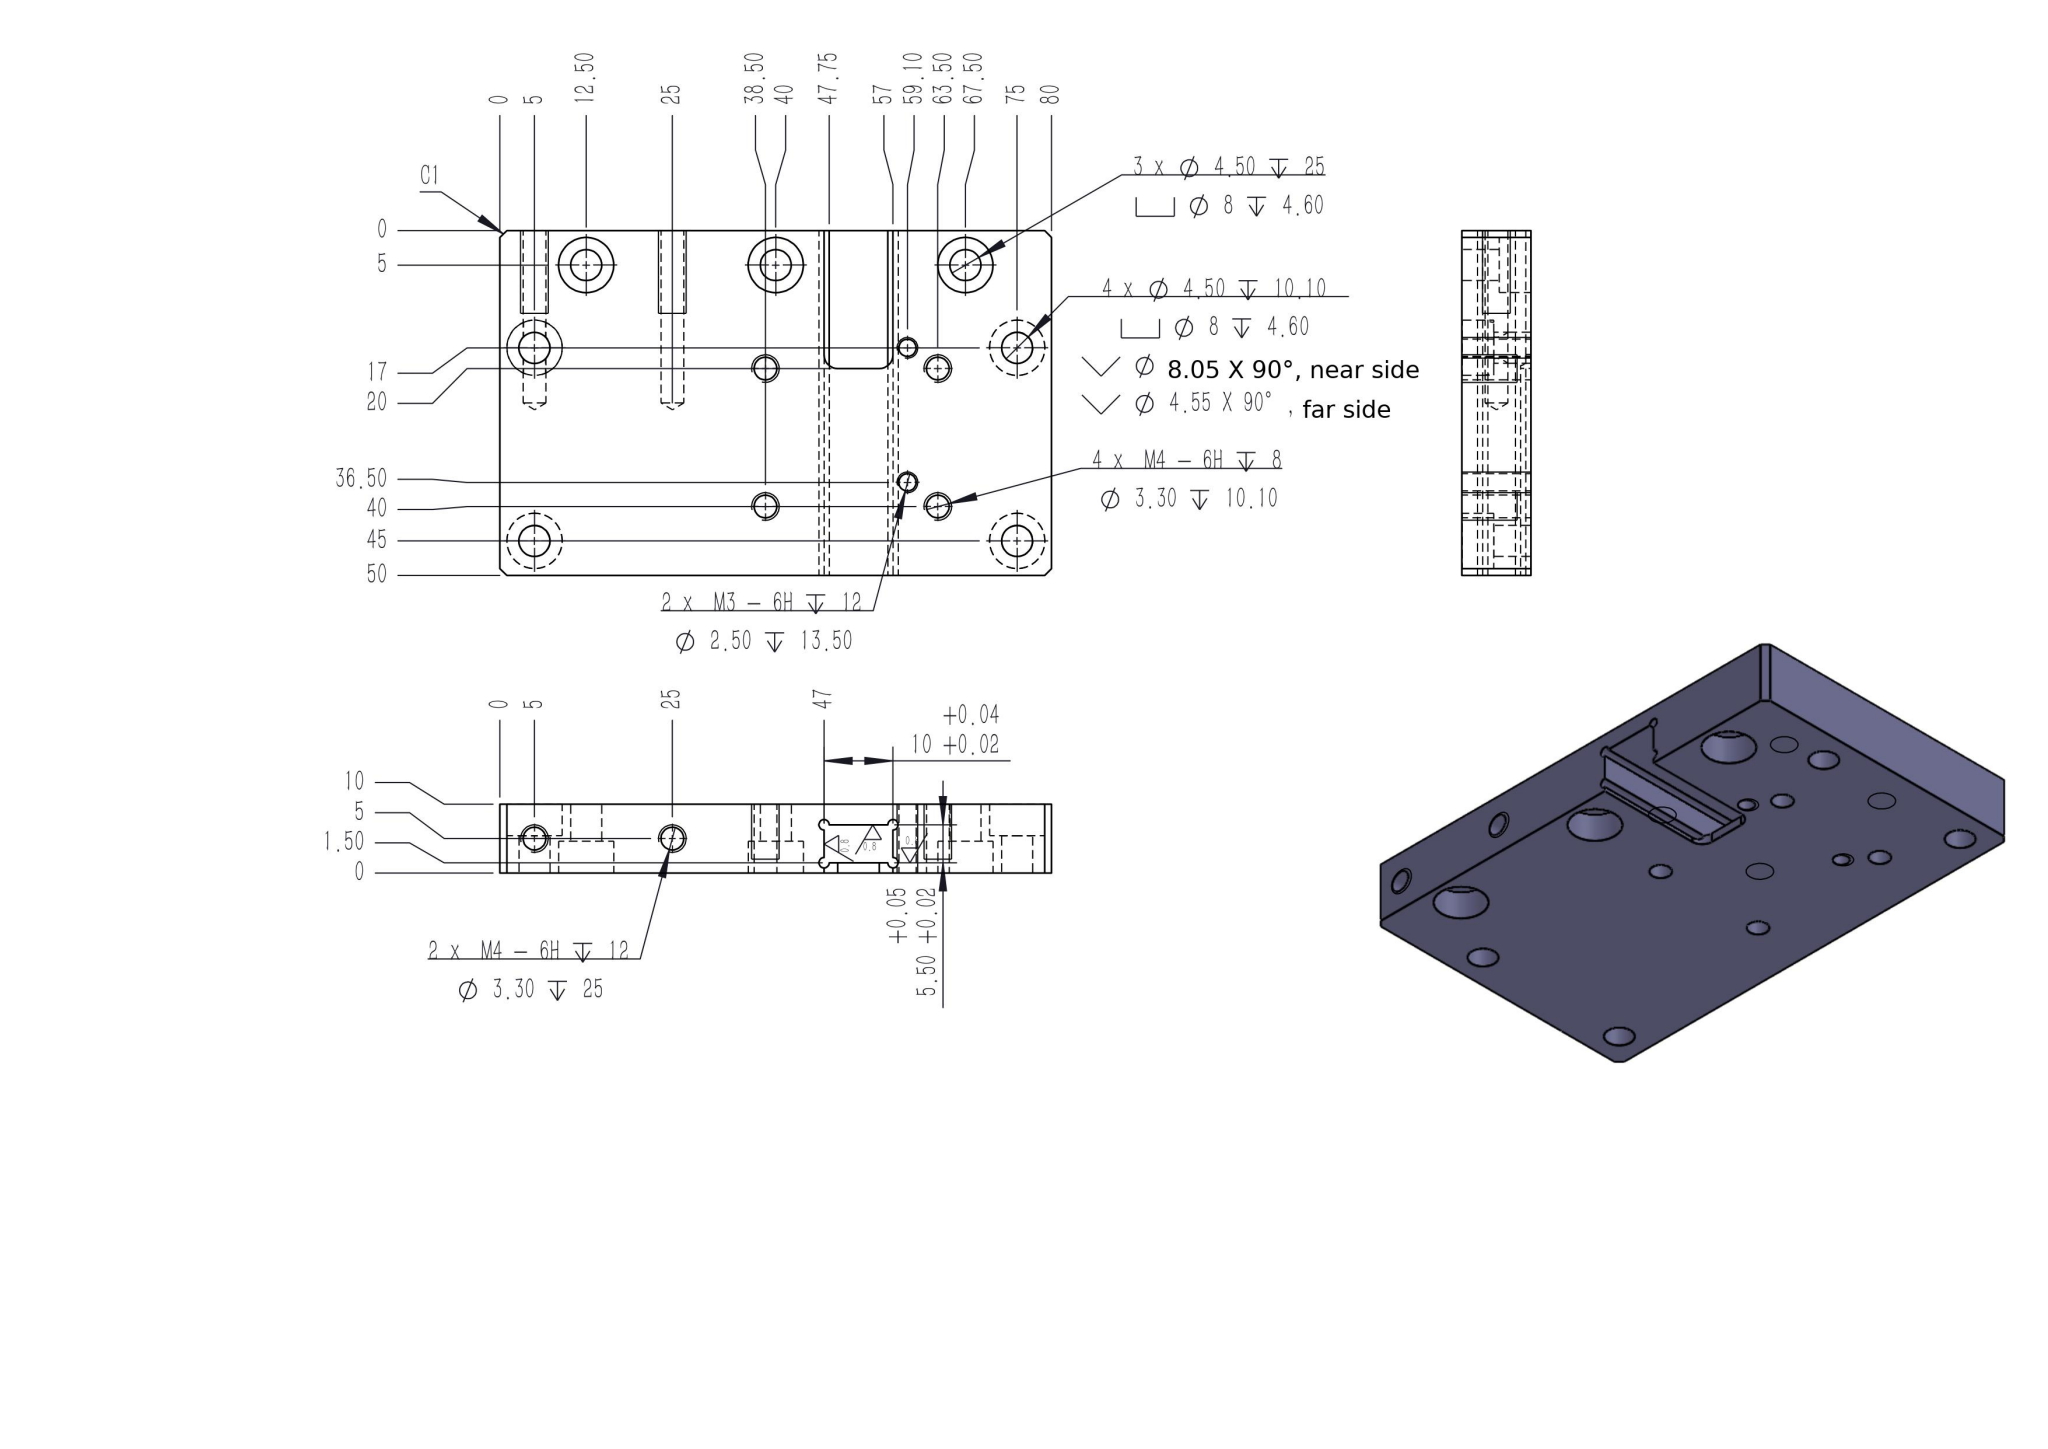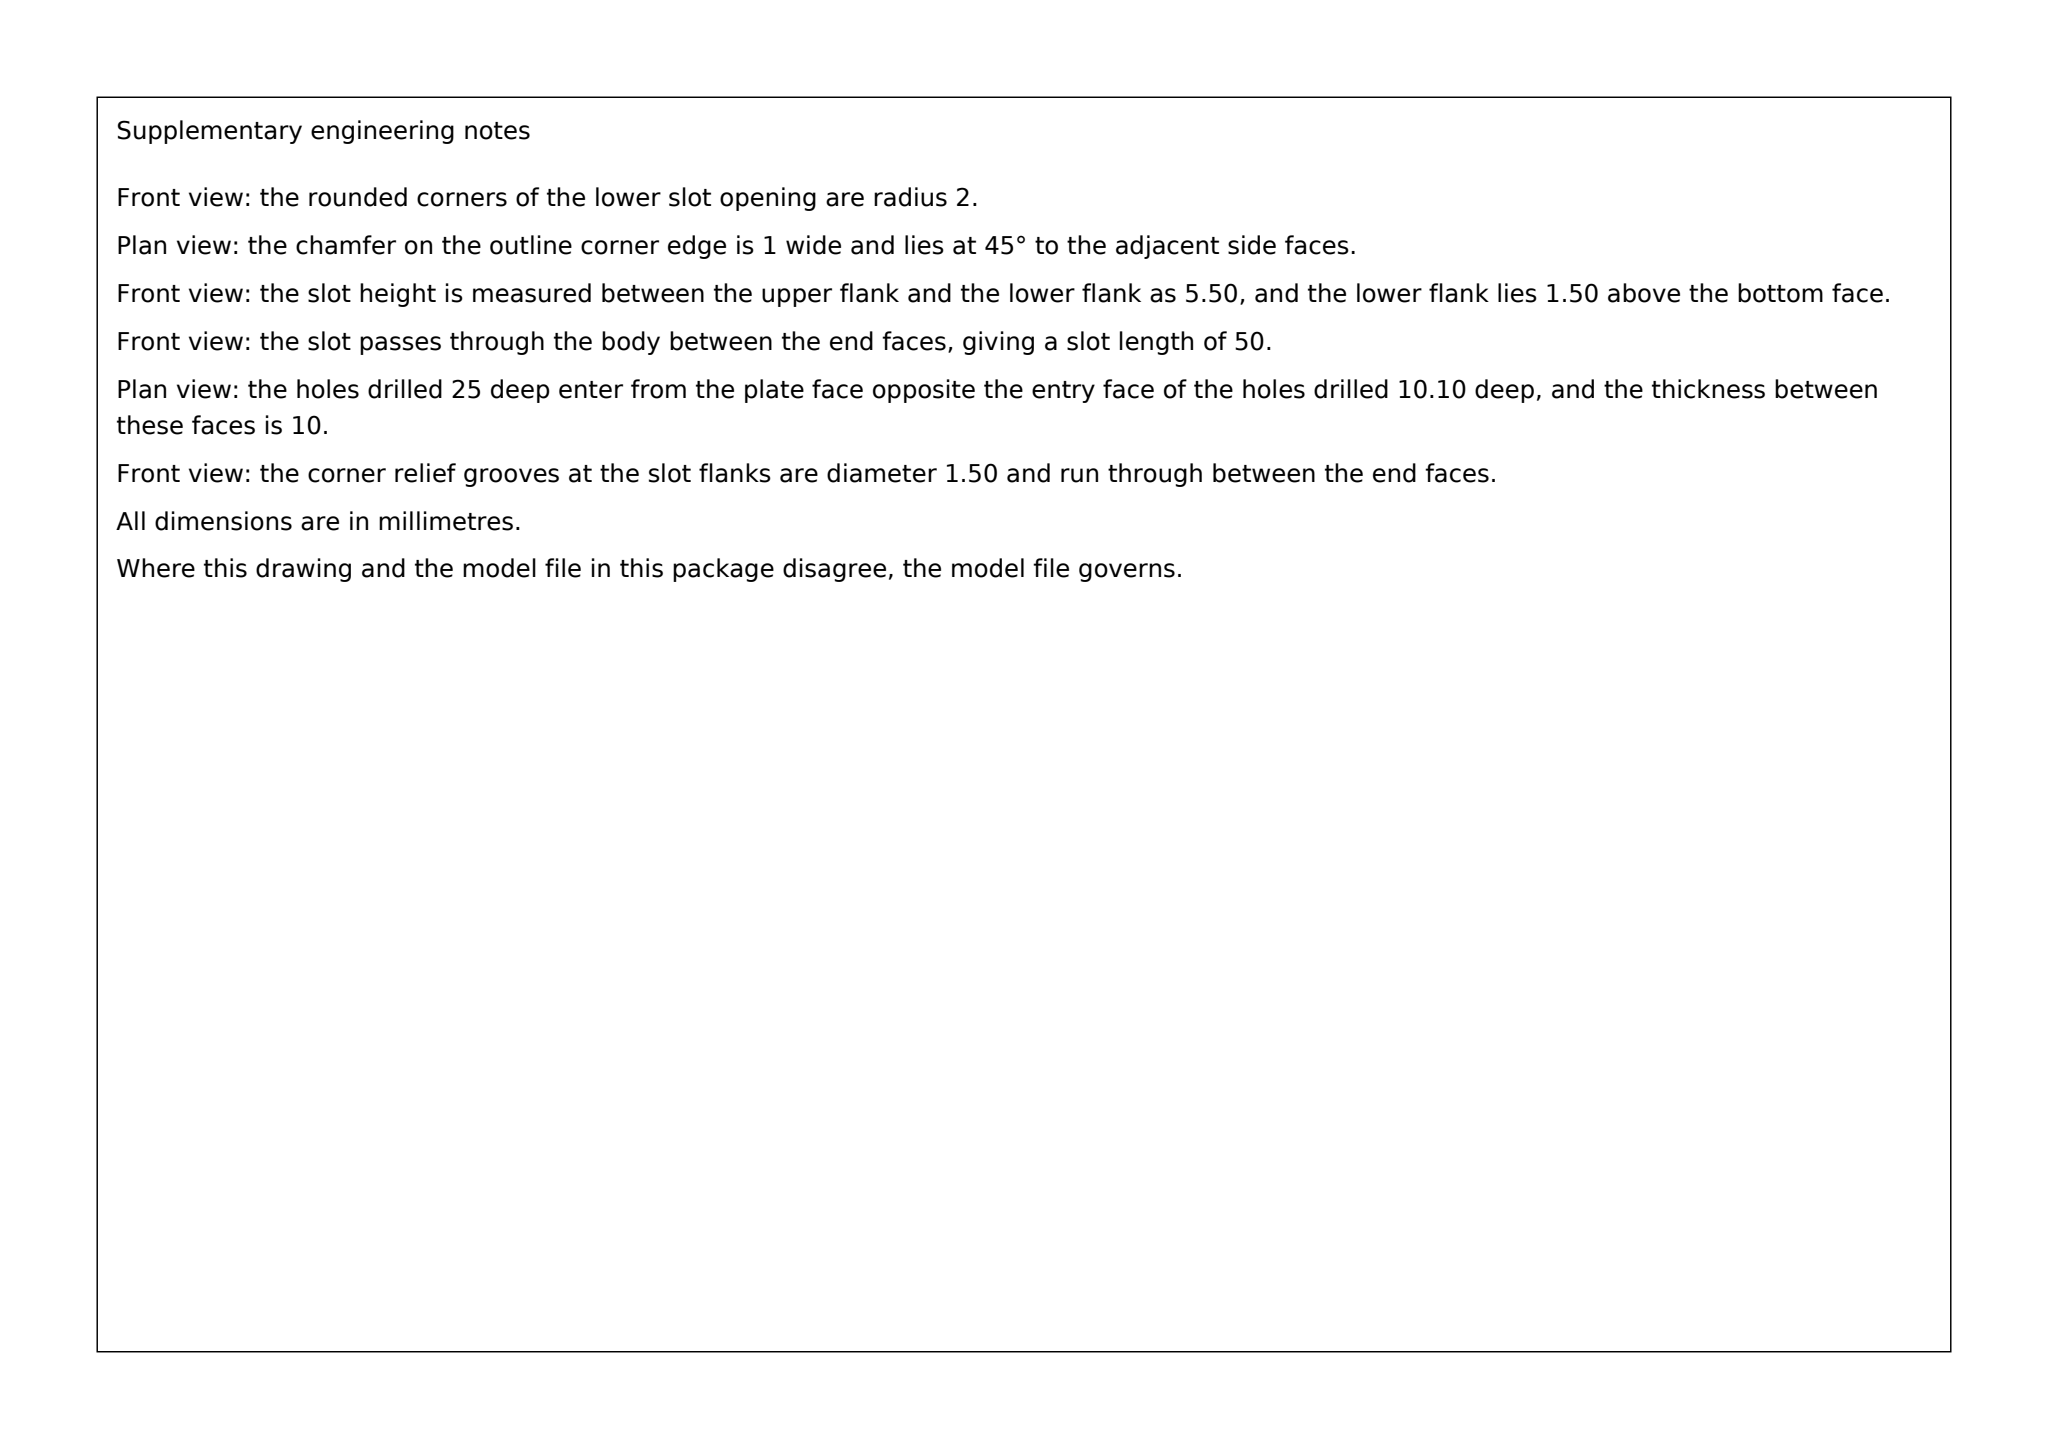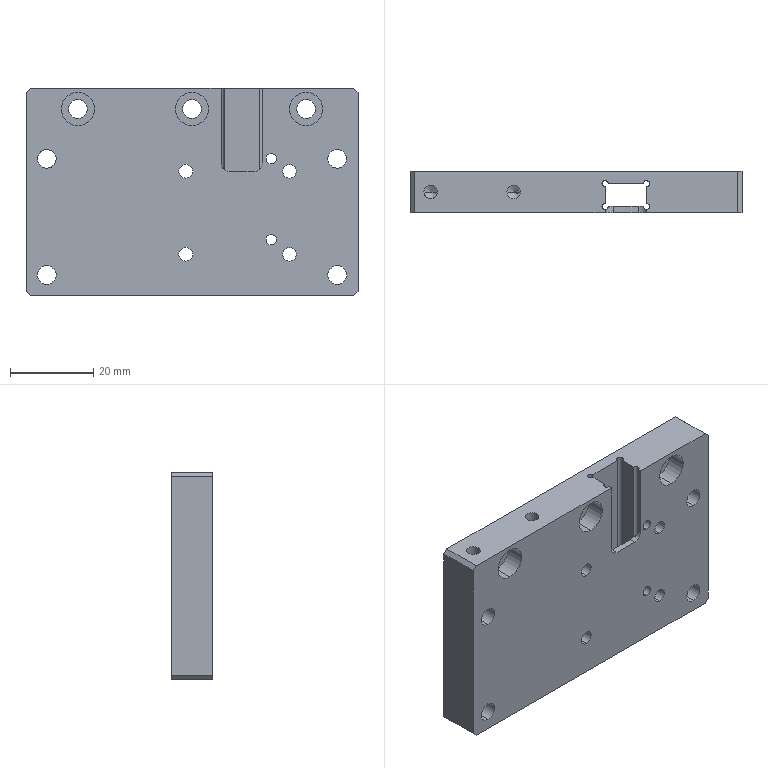Part | SolidWorks | mm | 1 solid | 99 faces | box 80 x 10 x 50 mm | volume 33637 mm3 | cylinder 54 | plane 25 | cone 20 | commonest cylinder face diameters 3.3 x14 4.5 x14 8 x14 1.5 x6 2.5 x4 4 x2
Drawing notes:
4X C1 - ALL 4 CORNERS, FULL 10 THK | from the solid: 4 inclined planes 45deg, size 1 x 10 x 1 at corners (0,0,0),(0,0,49),(79,0,0),(79,0,49)
build123d program:
from build123d import *

# Parameters (mm, degrees)
SKETCH1_W                                         = 80
SKETCH1_H                                         = 50
BOSS_EXTRUDE1_DEPTH                               = 10
M4_TAPPED_HOLE1_D                                 = 3.3
M4_TAPPED_HOLE1_DEPTH                             = 25
M4_TAPPED_HOLE1_TIP                               = 0.9914
HOLE_SIZE_ACCORDING_TO_HEXAGON_SOCKET_D           = 4.5
HOLE_SIZE_ACCORDING_TO_HEXAGON_SOCKET_DEPTH       = 25
HOLE_SIZE_ACCORDING_TO_HEXAGON_SOCKET_CBORE_D     = 8
HOLE_SIZE_ACCORDING_TO_HEXAGON_SOCKET_CBORE_DEPTH = 4.6
HOLE_SIZE_ACCORDING_TO_HEXAGON_SOCKET_TIP         = 1.352
SKETCH6_W                                         = 10
SKETCH6_H                                         = 122.914
CUT_EXTRUDE1_DEPTH                                = 7
SKETCH8_W                                         = 10
SKETCH8_H                                         = 1.5
BOSS_EXTRUDE3_DEPTH                               = 30
FILLET1_R                                         = 2
SKETCH9_R                                         = 0.75
CUT_EXTRUDE2_DEPTH                                = 67
M3_TAPPED_HOLE1_D                                 = 2.5
M3_TAPPED_HOLE1_DEPTH                             = 13.5
M3_TAPPED_HOLE1_TIP                               = 0.7511
HOLE_SIZE_ACCORDING_TO_HEXAGON_SO_2_A_COUNT       = 2
HOLE_SIZE_ACCORDING_TO_HEXAGON_SO_2_A_PITCH       = 28
HOLE_SIZE_ACCORDING_TO_HEXAGON_SO_3_COUNT         = 2
HOLE_SIZE_ACCORDING_TO_HEXAGON_SO_3_PITCH         = 70
HOLE_SIZE_ACCORDING_TO_HEXAGON_SO_4_COUNT         = 2
HOLE_SIZE_ACCORDING_TO_HEXAGON_SO_4_PITCH         = 75.392
M4_TAPPED_HOLE2_D                                 = 3.3
M4_TAPPED_HOLE2_DEPTH                             = 10.1
M4_TAPPED_HOLE2_TIP                               = 0.9914
CHAMFER1_SIZE                                     = 1


with BuildPart() as part:
    # Sketch1 → Boss-Extrude1 (new body)
    with BuildSketch(Plane(origin=(0, 0, 0), x_dir=(1, 0, 0), z_dir=(0, 1, 0))):
        Rectangle(SKETCH1_W, SKETCH1_H)
    extrude(amount=BOSS_EXTRUDE1_DEPTH)

    # M4 Tapped Hole1
    with Locations(Plane.XY.offset(25)):
        with Locations((-15, 5), (-35, 5)):
            Hole(M4_TAPPED_HOLE1_D / 2, depth=M4_TAPPED_HOLE1_DEPTH)
            with Locations((0, 0, -(M4_TAPPED_HOLE1_DEPTH + M4_TAPPED_HOLE1_TIP / 2))):  # 118° drill point
                Cone(0, M4_TAPPED_HOLE1_D / 2, M4_TAPPED_HOLE1_TIP, mode=Mode.SUBTRACT)

    # Hole Size _ according to_ Hexagon Socket
    with Locations(Plane(origin=(0, 0, 0), x_dir=(-1, 0, 0), z_dir=(0, -1, 0))):
        with Locations((27.5, -20), (-27.5, -20), (0, -20)):
            CounterBoreHole(HOLE_SIZE_ACCORDING_TO_HEXAGON_SOCKET_D / 2, HOLE_SIZE_ACCORDING_TO_HEXAGON_SOCKET_CBORE_D / 2, HOLE_SIZE_ACCORDING_TO_HEXAGON_SOCKET_CBORE_DEPTH, depth=HOLE_SIZE_ACCORDING_TO_HEXAGON_SOCKET_DEPTH)
            with Locations((0, 0, -(HOLE_SIZE_ACCORDING_TO_HEXAGON_SOCKET_DEPTH + HOLE_SIZE_ACCORDING_TO_HEXAGON_SOCKET_TIP / 2))):  # 118° drill point
                Cone(0, HOLE_SIZE_ACCORDING_TO_HEXAGON_SOCKET_D / 2, HOLE_SIZE_ACCORDING_TO_HEXAGON_SOCKET_TIP, mode=Mode.SUBTRACT)

    # Sketch6 → Cut-Extrude1 (cut)
    with BuildSketch(Plane.XZ):
        with Locations((12, 25)):
            Rectangle(SKETCH6_W, SKETCH6_H)
    extrude(amount=-CUT_EXTRUDE1_DEPTH, mode=Mode.SUBTRACT)

    # Sketch8 → Boss-Extrude3 (add)
    with BuildSketch(Plane(origin=(0, 0, -25), x_dir=(-1, 0, 0), z_dir=(0, 0, -1))):
        with Locations((-12, 0.75)):
            Rectangle(SKETCH8_W, SKETCH8_H)
    extrude(amount=-BOSS_EXTRUDE3_DEPTH)

    # Fillet1
    fillet1_edges = [part.edges().sort_by_distance(p)[0] for p in [
        (17, 0.75, 5),
        (7, 0.75, 5),
    ]]
    fillet(fillet1_edges, radius=FILLET1_R)

    # Sketch9 → Cut-Extrude2 (cut)
    with BuildSketch(Plane(origin=(0, 0, -25), x_dir=(-1, 0, 0), z_dir=(0, 0, -1))):
        with Locations((-17, 7)):
            Circle(SKETCH9_R)
        with Locations((-7, 7)):
            Circle(SKETCH9_R)
        with Locations((-7, 1.5)):
            Circle(SKETCH9_R)
        with Locations((-17, 1.5)):
            Circle(SKETCH9_R)
    extrude(amount=-CUT_EXTRUDE2_DEPTH, mode=Mode.SUBTRACT)

    # M3 Tapped Hole1
    with Locations(Plane(origin=(0, 0, 0), x_dir=(-1, 0, 0), z_dir=(0, -1, 0))):
        with Locations((-19.1, -8), (-19.1, 11.5)):
            Hole(M3_TAPPED_HOLE1_D / 2, depth=M3_TAPPED_HOLE1_DEPTH)
            with Locations((0, 0, -(M3_TAPPED_HOLE1_DEPTH + M3_TAPPED_HOLE1_TIP / 2))):  # 118° drill point
                Cone(0, M3_TAPPED_HOLE1_D / 2, M3_TAPPED_HOLE1_TIP, mode=Mode.SUBTRACT)

    # Sketch12 → Hole Size _ according to_ Hexagon So 2 (revolve, cut)
    with BuildSketch(Plane(origin=(-35, 10, 8), x_dir=(0, 0, 1), z_dir=(1, 0, 0))):
        Polygon((0, 0), (0, 11.452), (2.25, 10.1), (2.25, 4.625), (2.275, 4.6), (4, 4.6), (4, 0.025), (4.025, 0), align=None)
    hole_size_according_to_hexagon_so_2 = revolve(axis=Axis((-35, 16.35, 8), (0, -1, 0)), mode=Mode.SUBTRACT)

    # Hole Size _ according to_ Hexagon So 2 a: Hole Size _ according to_ Hexagon So 2 ×2
    with Locations(*[(0, 0, -i * HOLE_SIZE_ACCORDING_TO_HEXAGON_SO_2_A_PITCH) for i in range(1, HOLE_SIZE_ACCORDING_TO_HEXAGON_SO_2_A_COUNT)]):
        add(hole_size_according_to_hexagon_so_2, mode=Mode.SUBTRACT)

    # Hole Size _ according to_ Hexagon So 3: Hole Size _ according to_ Hexagon So 2 ×2
    with Locations(*[(i * HOLE_SIZE_ACCORDING_TO_HEXAGON_SO_3_PITCH, 0, 0) for i in range(1, HOLE_SIZE_ACCORDING_TO_HEXAGON_SO_3_COUNT)]):
        add(hole_size_according_to_hexagon_so_2, mode=Mode.SUBTRACT)

    # Hole Size _ according to_ Hexagon So 4: Hole Size _ according to_ Hexagon So 2 ×2
    with Locations(*[Vector(0.9285, 0, -0.3714) * (i * HOLE_SIZE_ACCORDING_TO_HEXAGON_SO_4_PITCH) for i in range(1, HOLE_SIZE_ACCORDING_TO_HEXAGON_SO_4_COUNT)]):
        add(hole_size_according_to_hexagon_so_2, mode=Mode.SUBTRACT)

    # M4 Tapped Hole2
    with Locations(Plane(origin=(0, 10, 0), x_dir=(1, 0, 0), z_dir=(0, 1, 0))):
        with Locations((-1.5, 15), (23.5, 15), (23.5, -5), (-1.5, -5)):
            Hole(M4_TAPPED_HOLE2_D / 2, depth=M4_TAPPED_HOLE2_DEPTH)
            with Locations((0, 0, -(M4_TAPPED_HOLE2_DEPTH + M4_TAPPED_HOLE2_TIP / 2))):  # 118° drill point
                Cone(0, M4_TAPPED_HOLE2_D / 2, M4_TAPPED_HOLE2_TIP, mode=Mode.SUBTRACT)

    # Chamfer1
    chamfer1_edges = [part.edges().sort_by_distance(p)[0] for p in [
        (40, 5, 25),
        (-40, 5, 25),
        (-40, 5, -25),
        (40, 5, -25),
    ]]
    chamfer(chamfer1_edges, length=CHAMFER1_SIZE)


solid = part.part